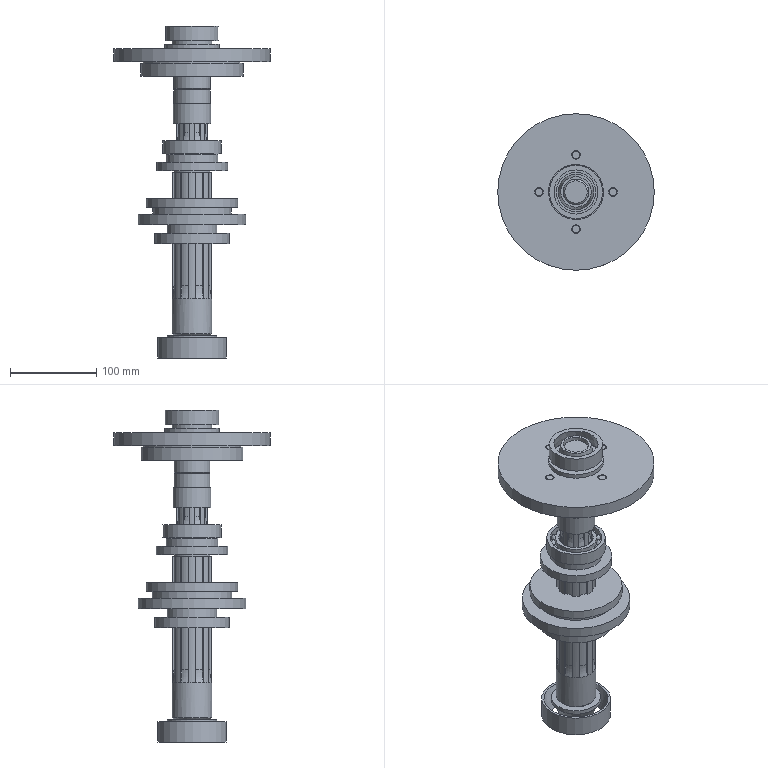Assembly | NX | mm | 13 component files | 17 solids | 447 faces | box 181.5 x 181.5 x 385.26 mm | volume 1521166 mm3 | plane 221 | cylinder 160 | torus 32 | cone 18 | sphere 16 | commonest cylinder face diameters 46 x33 42.5 x32 32 x24 36 x17 15 x8 8.5 x8 30 x4 10 x4
Bill of materials:
unnamed part 1 | 1 |  | Stepped flanged ring: a wide thin circular flange with a smaller, taller cylindrical hub on one face, and a through bore with eight evenly spaced rectangular internal notches (splined/keyed bore).
unnamed part 2 | 1 |  | Two concentric rings with a visible annular gap between them: a taller outer cylindrical ring, and an inner ring with a tapered (conical) outer surface whose short cylindrical section sticks out past one face of the outer ring.
unnamed part 3 | 1 |  | Ball-bearing-like body: an outer ring and an inner ring of equal width, with a single row of 16 spheres in the annular space between them and no visible cage.
unnamed part 4 | 1 |  | Long, slender stepped round shaft with several diameter sections, lengthwise splines or flutes on two of them, and smaller plain journal ends with narrow circumferential grooves.
unnamed part 5 | 1 |  | Thick-walled cylindrical sleeve whose outside diameter steps once: a slightly smaller upper section with a chamfered top edge, and a larger lower section. The through bore has eight evenly spaced rectangular internal notches.
unnamed part 6 | 1 |  | Stacked hub of coaxial discs: a top disc, a short smaller-diameter step, the largest-diameter flange, a narrow reduced neck, and a lower disc. A small central through bore has eight small notches.
unnamed part 7 | 1 |  | Thin circular disc with a central hub: a short boss on the top face and a two-step boss on the underside, the lowest step having a chamfered end. There is a central bore with eight notches, a shallow circular recess or ridge around the bore on the top face, and four small through-holes evenly spaced on a circle.
unnamed part 8 | 1 |  | Flat annular plate: a constant-thickness ring with a large central round hole and four small round through-holes evenly spaced on a circle between the bore and the outer edge.
unnamed part 9 | 1 |  | Two concentric rings: an outer cylindrical ring with a conical (tapered) inner surface, and an inner ring with a tapered outer surface and a plain bore. The inner ring's flat top face stands slightly proud of the outer ring.
unnamed part 10 | 4 |  | Headed cylindrical pin: a plain round shank with a short, larger-diameter flat head at one end, and a small rectangular radial notch cut into the head's rim.
Mates:
1. parallel | SLCLZY 1 face | assembly face
2. parallel | ZYC44 1 face | assembly face
3. concentric | ZYC44 1 edge | assembly edge
4. parallel | ZYC44 1 face | assembly face
5. distance | ZYC63 1 | assembly face
6. parallel | ZYC63 1 face | assembly face
7. touch align | ZYC63 1 face | assembly edge
8. concentric | ZYC50 1 edge | ZYC63 1
9. concentric | ZYC50 1 edge | ZYC63 1 edge
10. parallel | ZYC20 1 face | assembly face
11. concentric | ZYC20 1 edge | ZYC63 1 edge
12. concentric | ZYD 4 edge | ZYC63 1
13. concentric | ZYD 3 edge | ZYC63 1
14. concentric | ZYD 2 edge | ZYC63 1 edge
15. concentric | ZYD 1 edge | ZYC63 1
16. touch align | gundongzhoucheng 1 face | assembly face
17. touch align | gundongzhoucheng 1 face | ZYC44 1 face
18. parallel | assembly nxobject | assembly face
19. touch align | gunzizhouchou 1 face | assembly face
20. touch align | gunzizhouchou 1 face | assembly face
21. touch align | gunzizgouchou2 1 face | ZYC63 1 face